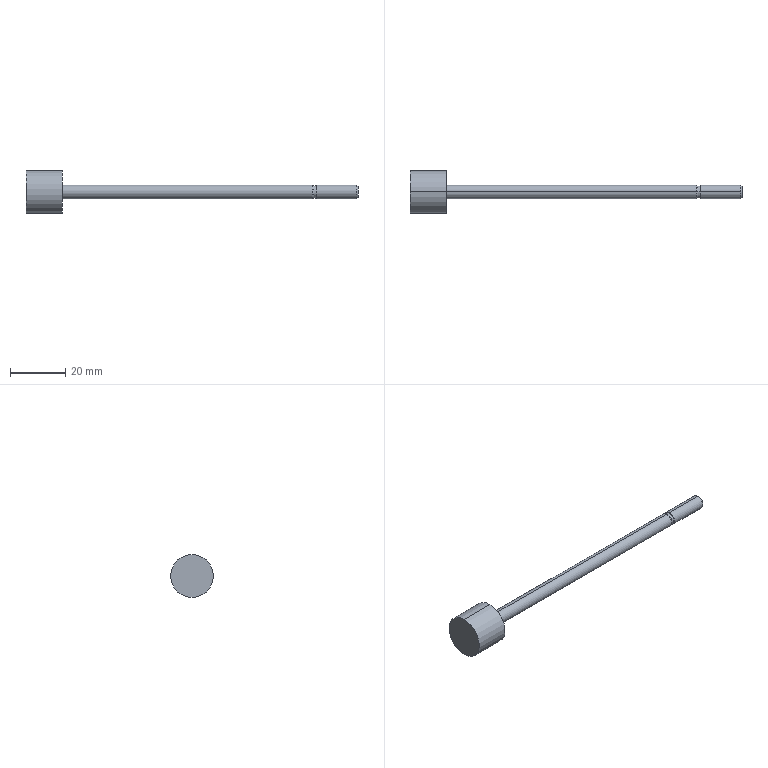Component | SolidWorks | 17268PB16x60SU(58)+(CS1-M-2)-1_1726816PB60URod-1 | 1 solid | 16 faces | box 120.36 x 15.5 x 15.5 mm | volume 4587 mm3 | cylinder 8 | cone 4 | plane 4 | commonest cylinder face diameters 5 x4 15.5 x2 4.38 x2
build123d program:
from build123d import *


with BuildPart() as part:
    # Sketch1 → Revolve1 (revolve)
    with BuildSketch(Plane.XY, mode=Mode.PRIVATE) as revolve1_sk:
        Polygon((0, 0), (0, 2.01), (0.4905, 2.5), (15, 2.5), (15, 2.19), (16, 2.19), (16.5, 2.5), (107.16, 2.5), (107.16, 7.75), (120.36, 7.75), (120.36, 0), align=None)
    revolve(revolve1_sk.sketch.rotate(Axis((120.36, 0, 0), (-1, 0, 0)), 270), axis=Axis((120.36, 0, 0), (-1, 0, 0)))


solid = part.part

# Placed as in the assembly
solid = solid.moved(Location((7, -27.579, 21.5), (-180, 0, 180)))
STEP:
#1=CARTESIAN_POINT('',(-4.463,-1.086,0.5413));
#2=VERTEX_POINT('',#1);
#3=CARTESIAN_POINT('',(-4.463,-1.086,1.152));
#4=VERTEX_POINT('',#3);
#5=CARTESIAN_POINT('',(-4.463,-1.086,0.8465));
#6=DIRECTION('',(1.,-0.,-0.));
#7=DIRECTION('',(0.,0.,-1.));
#8=AXIS2_PLACEMENT_3D('',#5,#6,#7);
#9=CIRCLE('',#8,0.3051);
#10=EDGE_CURVE('',#2,#4,#9,.T.);
#11=ORIENTED_EDGE('',*,*,#10,.T.);
#12=CARTESIAN_POINT('',(-3.943,-1.086,1.152));
#13=VERTEX_POINT('',#12);
#14=CARTESIAN_POINT('',(-4.463,-1.086,1.152));
#15=DIRECTION('',(1.,-0.,-0.));
#16=VECTOR('',#15,39.37);
#17=LINE('',#14,#16);
#18=EDGE_CURVE('',#4,#13,#17,.T.);
#19=ORIENTED_EDGE('',*,*,#18,.T.);
#20=CARTESIAN_POINT('',(-3.943,-1.086,0.5413));
#21=VERTEX_POINT('',#20);
#22=CARTESIAN_POINT('',(-3.943,-1.086,0.8465));
#23=DIRECTION('',(1.,-0.,-0.));
#24=DIRECTION('',(0.,0.,-1.));
#25=AXIS2_PLACEMENT_3D('',#22,#23,#24);
#26=CIRCLE('',#25,0.3051);
#27=EDGE_CURVE('',#21,#13,#26,.T.);
#28=ORIENTED_EDGE('',*,*,#27,.F.);
#29=CARTESIAN_POINT('',(-4.463,-1.086,0.5413));
#30=DIRECTION('',(1.,-0.,-0.));
#31=VECTOR('',#30,39.37);
#32=LINE('',#29,#31);
#33=EDGE_CURVE('',#2,#21,#32,.T.);
#34=ORIENTED_EDGE('',*,*,#33,.F.);
#35=EDGE_LOOP('',(#11,#19,#28,#34));
#36=FACE_OUTER_BOUND('',#35,.T.);
#37=CARTESIAN_POINT('',(-4.463,-1.086,0.8465));
#38=DIRECTION('',(1.,-0.,-0.));
#39=DIRECTION('',(0.,0.,-1.));
#40=AXIS2_PLACEMENT_3D('',#37,#38,#39);
#41=CYLINDRICAL_SURFACE('',#40,0.3051);
#42=ADVANCED_FACE('',(#36),#41,.T.);
#43=CARTESIAN_POINT('',(-3.943,-1.086,0.748));
#44=VERTEX_POINT('',#43);
#45=CARTESIAN_POINT('',(-3.943,-1.086,0.9449));
#46=VERTEX_POINT('',#45);
#47=CARTESIAN_POINT('',(-3.943,-1.086,0.8465));
#48=DIRECTION('',(1.,-0.,-0.));
#49=DIRECTION('',(0.,0.,-1.));
#50=AXIS2_PLACEMENT_3D('',#47,#48,#49);
#51=CIRCLE('',#50,0.09843);
#52=EDGE_CURVE('',#44,#46,#51,.T.);
#53=ORIENTED_EDGE('',*,*,#52,.T.);
#54=CARTESIAN_POINT('',(-0.374,-1.086,0.9449));
#55=VERTEX_POINT('',#54);
#56=CARTESIAN_POINT('',(-4.463,-1.086,0.9449));
#57=DIRECTION('',(1.,-0.,-0.));
#58=VECTOR('',#57,39.37);
#59=LINE('',#56,#58);
#60=EDGE_CURVE('',#46,#55,#59,.T.);
#61=ORIENTED_EDGE('',*,*,#60,.T.);
#62=CARTESIAN_POINT('',(-0.374,-1.086,0.748));
#63=VERTEX_POINT('',#62);
#64=CARTESIAN_POINT('',(-0.374,-1.086,0.8465));
#65=DIRECTION('',(1.,-0.,-0.));
#66=DIRECTION('',(0.,0.,-1.));
#67=AXIS2_PLACEMENT_3D('',#64,#65,#66);
#68=CIRCLE('',#67,0.09843);
#69=EDGE_CURVE('',#63,#55,#68,.T.);
#70=ORIENTED_EDGE('',*,*,#69,.F.);
#71=CARTESIAN_POINT('',(-4.463,-1.086,0.748));
#72=DIRECTION('',(1.,-0.,-0.));
#73=VECTOR('',#72,39.37);
#74=LINE('',#71,#73);
#75=EDGE_CURVE('',#44,#63,#74,.T.);
#76=ORIENTED_EDGE('',*,*,#75,.F.);
#77=EDGE_LOOP('',(#53,#61,#70,#76));
#78=FACE_OUTER_BOUND('',#77,.T.);
#79=CARTESIAN_POINT('',(-4.463,-1.086,0.8465));
#80=DIRECTION('',(1.,-0.,-0.));
#81=DIRECTION('',(0.,0.,-1.));
#82=AXIS2_PLACEMENT_3D('',#79,#80,#81);
#83=CYLINDRICAL_SURFACE('',#82,0.09843);
#84=ADVANCED_FACE('',(#78),#83,.T.);
#85=CARTESIAN_POINT('',(-0.3543,-1.086,0.7602));
#86=VERTEX_POINT('',#85);
#87=CARTESIAN_POINT('',(-0.3543,-1.086,0.9327));
#88=VERTEX_POINT('',#87);
#89=CARTESIAN_POINT('',(-0.3543,-1.086,0.8465));
#90=DIRECTION('',(1.,-0.,-0.));
#91=DIRECTION('',(0.,0.,-1.));
#92=AXIS2_PLACEMENT_3D('',#89,#90,#91);
#93=CIRCLE('',#92,0.08622);
#94=EDGE_CURVE('',#86,#88,#93,.T.);
#95=ORIENTED_EDGE('',*,*,#94,.F.);
#96=CARTESIAN_POINT('',(-0.374,-1.086,0.748));
#97=DIRECTION('',(-0.8499,0.,-0.5269));
#98=VECTOR('',#97,39.37);
#99=LINE('',#96,#98);
#100=EDGE_CURVE('',#86,#63,#99,.T.);
#101=ORIENTED_EDGE('',*,*,#100,.T.);
#102=ORIENTED_EDGE('',*,*,#69,.T.);
#103=CARTESIAN_POINT('',(-0.374,-1.086,0.9449));
#104=DIRECTION('',(-0.8499,0.,0.5269));
#105=VECTOR('',#104,39.37);
#106=LINE('',#103,#105);
#107=EDGE_CURVE('',#88,#55,#106,.T.);
#108=ORIENTED_EDGE('',*,*,#107,.F.);
#109=EDGE_LOOP('',(#95,#101,#102,#108));
#110=FACE_OUTER_BOUND('',#109,.T.);
#111=CARTESIAN_POINT('',(-0.374,-1.086,0.8465));
#112=DIRECTION('',(-1.,0.,0.));
#113=DIRECTION('',(0.,0.,1.));
#114=AXIS2_PLACEMENT_3D('',#111,#112,#113);
#115=CONICAL_SURFACE('',#114,0.09843,0.555);
#116=ADVANCED_FACE('',(#110),#115,.T.);
#117=ORIENTED_EDGE('',*,*,#94,.T.);
#118=CARTESIAN_POINT('',(-0.315,-1.086,0.9327));
#119=VERTEX_POINT('',#118);
#120=CARTESIAN_POINT('',(-4.463,-1.086,0.9327));
#121=DIRECTION('',(1.,-0.,-0.));
#122=VECTOR('',#121,39.37);
#123=LINE('',#120,#122);
#124=EDGE_CURVE('',#88,#119,#123,.T.);
#125=ORIENTED_EDGE('',*,*,#124,.T.);
#126=CARTESIAN_POINT('',(-0.315,-1.086,0.7602));
#127=VERTEX_POINT('',#126);
#128=CARTESIAN_POINT('',(-0.315,-1.086,0.8465));
#129=DIRECTION('',(1.,-0.,-0.));
#130=DIRECTION('',(0.,0.,-1.));
#131=AXIS2_PLACEMENT_3D('',#128,#129,#130);
#132=CIRCLE('',#131,0.08622);
#133=EDGE_CURVE('',#127,#119,#132,.T.);
#134=ORIENTED_EDGE('',*,*,#133,.F.);
#135=CARTESIAN_POINT('',(-4.463,-1.086,0.7602));
#136=DIRECTION('',(1.,-0.,-0.));
#137=VECTOR('',#136,39.37);
#138=LINE('',#135,#137);
#139=EDGE_CURVE('',#86,#127,#138,.T.);
#140=ORIENTED_EDGE('',*,*,#139,.F.);
#141=EDGE_LOOP('',(#117,#125,#134,#140));
#142=FACE_OUTER_BOUND('',#141,.T.);
#143=CARTESIAN_POINT('',(-4.463,-1.086,0.8465));
#144=DIRECTION('',(1.,-0.,-0.));
#145=DIRECTION('',(0.,0.,-1.));
#146=AXIS2_PLACEMENT_3D('',#143,#144,#145);
#147=CYLINDRICAL_SURFACE('',#146,0.08622);
#148=ADVANCED_FACE('',(#142),#147,.T.);
#149=CARTESIAN_POINT('',(-0.315,-1.086,0.748));
#150=VERTEX_POINT('',#149);
#151=CARTESIAN_POINT('',(-0.315,-1.086,0.9449));
#152=VERTEX_POINT('',#151);
#153=CARTESIAN_POINT('',(-0.315,-1.086,0.8465));
#154=DIRECTION('',(1.,-0.,-0.));
#155=DIRECTION('',(0.,0.,-1.));
#156=AXIS2_PLACEMENT_3D('',#153,#154,#155);
#157=CIRCLE('',#156,0.09843);
#158=EDGE_CURVE('',#150,#152,#157,.T.);
#159=ORIENTED_EDGE('',*,*,#158,.T.);
#160=CARTESIAN_POINT('',(0.2563,-1.086,0.9449));
#161=VERTEX_POINT('',#160);
#162=CARTESIAN_POINT('',(-4.463,-1.086,0.9449));
#163=DIRECTION('',(1.,-0.,-0.));
#164=VECTOR('',#163,39.37);
#165=LINE('',#162,#164);
#166=EDGE_CURVE('',#152,#161,#165,.T.);
#167=ORIENTED_EDGE('',*,*,#166,.T.);
#168=CARTESIAN_POINT('',(0.2563,-1.086,0.748));
#169=VERTEX_POINT('',#168);
#170=CARTESIAN_POINT('',(0.2563,-1.086,0.8465));
#171=DIRECTION('',(1.,-0.,-0.));
#172=DIRECTION('',(0.,0.,-1.));
#173=AXIS2_PLACEMENT_3D('',#170,#171,#172);
#174=CIRCLE('',#173,0.09843);
#175=EDGE_CURVE('',#169,#161,#174,.T.);
#176=ORIENTED_EDGE('',*,*,#175,.F.);
#177=CARTESIAN_POINT('',(-4.463,-1.086,0.748));
#178=DIRECTION('',(1.,-0.,-0.));
#179=VECTOR('',#178,39.37);
#180=LINE('',#177,#179);
#181=EDGE_CURVE('',#150,#169,#180,.T.);
#182=ORIENTED_EDGE('',*,*,#181,.F.);
#183=EDGE_LOOP('',(#159,#167,#176,#182));
#184=FACE_OUTER_BOUND('',#183,.T.);
#185=CARTESIAN_POINT('',(-4.463,-1.086,0.8465));
#186=DIRECTION('',(1.,-0.,-0.));
#187=DIRECTION('',(0.,0.,-1.));
#188=AXIS2_PLACEMENT_3D('',#185,#186,#187);
#189=CYLINDRICAL_SURFACE('',#188,0.09843);
#190=ADVANCED_FACE('',(#184),#189,.T.);
#191=CARTESIAN_POINT('',(0.2756,-1.086,0.7673));
#192=VERTEX_POINT('',#191);
#193=CARTESIAN_POINT('',(0.2756,-1.086,0.9256));
#194=VERTEX_POINT('',#193);
#195=CARTESIAN_POINT('',(0.2756,-1.086,0.8465));
#196=DIRECTION('',(1.,-0.,-0.));
#197=DIRECTION('',(0.,0.,-1.));
#198=AXIS2_PLACEMENT_3D('',#195,#196,#197);
#199=CIRCLE('',#198,0.07911);
#200=EDGE_CURVE('',#192,#194,#199,.T.);
#201=ORIENTED_EDGE('',*,*,#200,.F.);
#202=CARTESIAN_POINT('',(0.2563,-1.086,0.748));
#203=DIRECTION('',(-0.7071,0.,-0.7071));
#204=VECTOR('',#203,39.37);
#205=LINE('',#202,#204);
#206=EDGE_CURVE('',#192,#169,#205,.T.);
#207=ORIENTED_EDGE('',*,*,#206,.T.);
#208=ORIENTED_EDGE('',*,*,#175,.T.);
#209=CARTESIAN_POINT('',(0.2563,-1.086,0.9449));
#210=DIRECTION('',(-0.7071,0.,0.7071));
#211=VECTOR('',#210,39.37);
#212=LINE('',#209,#211);
#213=EDGE_CURVE('',#194,#161,#212,.T.);
#214=ORIENTED_EDGE('',*,*,#213,.F.);
#215=EDGE_LOOP('',(#201,#207,#208,#214));
#216=FACE_OUTER_BOUND('',#215,.T.);
#217=CARTESIAN_POINT('',(0.2563,-1.086,0.8465));
#218=DIRECTION('',(-1.,0.,0.));
#219=DIRECTION('',(0.,0.,1.));
#220=AXIS2_PLACEMENT_3D('',#217,#218,#219);
#221=CONICAL_SURFACE('',#220,0.09843,0.7854);
#222=ADVANCED_FACE('',(#216),#221,.T.);
#223=CARTESIAN_POINT('',(0.2756,-1.086,0.8465));
#224=DIRECTION('',(1.,-0.,-0.));
#225=DIRECTION('',(0.,0.,-1.));
#226=AXIS2_PLACEMENT_3D('',#223,#224,#225);
#227=CIRCLE('',#226,0.07911);
#228=EDGE_CURVE('',#194,#192,#227,.T.);
#229=ORIENTED_EDGE('',*,*,#228,.T.);
#230=ORIENTED_EDGE('',*,*,#200,.T.);
#231=EDGE_LOOP('',(#229,#230));
#232=FACE_OUTER_BOUND('',#231,.T.);
#233=CARTESIAN_POINT('',(0.2756,-1.086,0.8465));
#234=DIRECTION('',(-1.,0.,0.));
#235=DIRECTION('',(0.,0.,1.));
#236=AXIS2_PLACEMENT_3D('',#233,#234,#235);
#237=PLANE('',#236);
#238=ADVANCED_FACE('',(#232),#237,.F.);
#239=ORIENTED_EDGE('',*,*,#206,.F.);
#240=ORIENTED_EDGE('',*,*,#228,.F.);
#241=ORIENTED_EDGE('',*,*,#213,.T.);
#242=CARTESIAN_POINT('',(0.2563,-1.086,0.8465));
#243=DIRECTION('',(1.,-0.,-0.));
#244=DIRECTION('',(0.,0.,-1.));
#245=AXIS2_PLACEMENT_3D('',#242,#243,#244);
#246=CIRCLE('',#245,0.09843);
#247=EDGE_CURVE('',#161,#169,#246,.T.);
#248=ORIENTED_EDGE('',*,*,#247,.T.);
#249=EDGE_LOOP('',(#239,#240,#241,#248));
#250=FACE_OUTER_BOUND('',#249,.T.);
#251=CARTESIAN_POINT('',(0.2563,-1.086,0.8465));
#252=DIRECTION('',(-1.,0.,0.));
#253=DIRECTION('',(0.,0.,1.));
#254=AXIS2_PLACEMENT_3D('',#251,#252,#253);
#255=CONICAL_SURFACE('',#254,0.09843,0.7854);
#256=ADVANCED_FACE('',(#250),#255,.T.);
#257=ORIENTED_EDGE('',*,*,#166,.F.);
#258=CARTESIAN_POINT('',(-0.315,-1.086,0.8465));
#259=DIRECTION('',(1.,-0.,-0.));
#260=DIRECTION('',(0.,0.,-1.));
#261=AXIS2_PLACEMENT_3D('',#258,#259,#260);
#262=CIRCLE('',#261,0.09843);
#263=EDGE_CURVE('',#152,#150,#262,.T.);
#264=ORIENTED_EDGE('',*,*,#263,.T.);
#265=ORIENTED_EDGE('',*,*,#181,.T.);
#266=ORIENTED_EDGE('',*,*,#247,.F.);
#267=EDGE_LOOP('',(#257,#264,#265,#266));
#268=FACE_OUTER_BOUND('',#267,.T.);
#269=CARTESIAN_POINT('',(-4.463,-1.086,0.8465));
#270=DIRECTION('',(1.,-0.,-0.));
#271=DIRECTION('',(0.,0.,-1.));
#272=AXIS2_PLACEMENT_3D('',#269,#270,#271);
#273=CYLINDRICAL_SURFACE('',#272,0.09843);
#274=ADVANCED_FACE('',(#268),#273,.T.);
#275=ORIENTED_EDGE('',*,*,#158,.F.);
#276=ORIENTED_EDGE('',*,*,#263,.F.);
#277=EDGE_LOOP('',(#275,#276));
#278=FACE_OUTER_BOUND('',#277,.T.);
#279=ORIENTED_EDGE('',*,*,#133,.T.);
#280=CARTESIAN_POINT('',(-0.315,-1.086,0.8465));
#281=DIRECTION('',(1.,-0.,-0.));
#282=DIRECTION('',(0.,0.,-1.));
#283=AXIS2_PLACEMENT_3D('',#280,#281,#282);
#284=CIRCLE('',#283,0.08622);
#285=EDGE_CURVE('',#119,#127,#284,.T.);
#286=ORIENTED_EDGE('',*,*,#285,.T.);
#287=EDGE_LOOP('',(#279,#286));
#288=FACE_BOUND('',#287,.T.);
#289=CARTESIAN_POINT('',(-0.315,-0.9874,0.8465));
#290=DIRECTION('',(1.,-0.,-0.));
#291=DIRECTION('',(-0.,0.,-1.));
#292=AXIS2_PLACEMENT_3D('',#289,#290,#291);
#293=PLANE('',#292);
#294=ADVANCED_FACE('',(#278,#288),#293,.F.);
#295=ORIENTED_EDGE('',*,*,#124,.F.);
#296=CARTESIAN_POINT('',(-0.3543,-1.086,0.8465));
#297=DIRECTION('',(1.,-0.,-0.));
#298=DIRECTION('',(0.,0.,-1.));
#299=AXIS2_PLACEMENT_3D('',#296,#297,#298);
#300=CIRCLE('',#299,0.08622);
#301=EDGE_CURVE('',#88,#86,#300,.T.);
#302=ORIENTED_EDGE('',*,*,#301,.T.);
#303=ORIENTED_EDGE('',*,*,#139,.T.);
#304=ORIENTED_EDGE('',*,*,#285,.F.);
#305=EDGE_LOOP('',(#295,#302,#303,#304));
#306=FACE_OUTER_BOUND('',#305,.T.);
#307=CARTESIAN_POINT('',(-4.463,-1.086,0.8465));
#308=DIRECTION('',(1.,-0.,-0.));
#309=DIRECTION('',(0.,0.,-1.));
#310=AXIS2_PLACEMENT_3D('',#307,#308,#309);
#311=CYLINDRICAL_SURFACE('',#310,0.08622);
#312=ADVANCED_FACE('',(#306),#311,.T.);
#313=ORIENTED_EDGE('',*,*,#100,.F.);
#314=ORIENTED_EDGE('',*,*,#301,.F.);
#315=ORIENTED_EDGE('',*,*,#107,.T.);
#316=CARTESIAN_POINT('',(-0.374,-1.086,0.8465));
#317=DIRECTION('',(1.,-0.,-0.));
#318=DIRECTION('',(0.,0.,-1.));
#319=AXIS2_PLACEMENT_3D('',#316,#317,#318);
#320=CIRCLE('',#319,0.09843);
#321=EDGE_CURVE('',#55,#63,#320,.T.);
#322=ORIENTED_EDGE('',*,*,#321,.T.);
#323=EDGE_LOOP('',(#313,#314,#315,#322));
#324=FACE_OUTER_BOUND('',#323,.T.);
#325=CARTESIAN_POINT('',(-0.374,-1.086,0.8465));
#326=DIRECTION('',(-1.,0.,0.));
#327=DIRECTION('',(0.,0.,1.));
#328=AXIS2_PLACEMENT_3D('',#325,#326,#327);
#329=CONICAL_SURFACE('',#328,0.09843,0.555);
#330=ADVANCED_FACE('',(#324),#329,.T.);
#331=ORIENTED_EDGE('',*,*,#60,.F.);
#332=CARTESIAN_POINT('',(-3.943,-1.086,0.8465));
#333=DIRECTION('',(1.,-0.,-0.));
#334=DIRECTION('',(0.,0.,-1.));
#335=AXIS2_PLACEMENT_3D('',#332,#333,#334);
#336=CIRCLE('',#335,0.09843);
#337=EDGE_CURVE('',#46,#44,#336,.T.);
#338=ORIENTED_EDGE('',*,*,#337,.T.);
#339=ORIENTED_EDGE('',*,*,#75,.T.);
#340=ORIENTED_EDGE('',*,*,#321,.F.);
#341=EDGE_LOOP('',(#331,#338,#339,#340));
#342=FACE_OUTER_BOUND('',#341,.T.);
#343=CARTESIAN_POINT('',(-4.463,-1.086,0.8465));
#344=DIRECTION('',(1.,-0.,-0.));
#345=DIRECTION('',(0.,0.,-1.));
#346=AXIS2_PLACEMENT_3D('',#343,#344,#345);
#347=CYLINDRICAL_SURFACE('',#346,0.09843);
#348=ADVANCED_FACE('',(#342),#347,.T.);
#349=ORIENTED_EDGE('',*,*,#52,.F.);
#350=ORIENTED_EDGE('',*,*,#337,.F.);
#351=EDGE_LOOP('',(#349,#350));
#352=FACE_BOUND('',#351,.T.);
#353=ORIENTED_EDGE('',*,*,#27,.T.);
#354=CARTESIAN_POINT('',(-3.943,-1.086,0.8465));
#355=DIRECTION('',(1.,-0.,-0.));
#356=DIRECTION('',(0.,0.,-1.));
#357=AXIS2_PLACEMENT_3D('',#354,#355,#356);
#358=CIRCLE('',#357,0.3051);
#359=EDGE_CURVE('',#13,#21,#358,.T.);
#360=ORIENTED_EDGE('',*,*,#359,.T.);
#361=EDGE_LOOP('',(#353,#360));
#362=FACE_OUTER_BOUND('',#361,.T.);
#363=CARTESIAN_POINT('',(-3.943,-0.9874,0.8465));
#364=DIRECTION('',(-1.,0.,0.));
#365=DIRECTION('',(0.,0.,1.));
#366=AXIS2_PLACEMENT_3D('',#363,#364,#365);
#367=PLANE('',#366);
#368=ADVANCED_FACE('',(#352,#362),#367,.F.);
#369=ORIENTED_EDGE('',*,*,#18,.F.);
#370=CARTESIAN_POINT('',(-4.463,-1.086,0.8465));
#371=DIRECTION('',(1.,-0.,-0.));
#372=DIRECTION('',(0.,0.,-1.));
#373=AXIS2_PLACEMENT_3D('',#370,#371,#372);
#374=CIRCLE('',#373,0.3051);
#375=EDGE_CURVE('',#4,#2,#374,.T.);
#376=ORIENTED_EDGE('',*,*,#375,.T.);
#377=ORIENTED_EDGE('',*,*,#33,.T.);
#378=ORIENTED_EDGE('',*,*,#359,.F.);
#379=EDGE_LOOP('',(#369,#376,#377,#378));
#380=FACE_OUTER_BOUND('',#379,.T.);
#381=CARTESIAN_POINT('',(-4.463,-1.086,0.8465));
#382=DIRECTION('',(1.,-0.,-0.));
#383=DIRECTION('',(0.,0.,-1.));
#384=AXIS2_PLACEMENT_3D('',#381,#382,#383);
#385=CYLINDRICAL_SURFACE('',#384,0.3051);
#386=ADVANCED_FACE('',(#380),#385,.T.);
#387=ORIENTED_EDGE('',*,*,#10,.F.);
#388=ORIENTED_EDGE('',*,*,#375,.F.);
#389=EDGE_LOOP('',(#387,#388));
#390=FACE_OUTER_BOUND('',#389,.T.);
#391=CARTESIAN_POINT('',(-4.463,-0.7807,0.8465));
#392=DIRECTION('',(1.,-0.,-0.));
#393=DIRECTION('',(-0.,0.,-1.));
#394=AXIS2_PLACEMENT_3D('',#391,#392,#393);
#395=PLANE('',#394);
#396=ADVANCED_FACE('',(#390),#395,.F.);
#397=CLOSED_SHELL('',(#42,#84,#116,#148,#190,#222,#238,#256,#274,#294,#312,#330,#348,#368,#386,#396));
#398=MANIFOLD_SOLID_BREP('',#397);
#399=CARTESIAN_POINT('',(0.,0.,0.));
#400=DIRECTION('',(0.,0.,1.));
#401=DIRECTION('',(1.,0.,0.));
#402=AXIS2_PLACEMENT_3D('',#399,#400,#401);
#403=(LENGTH_UNIT()NAMED_UNIT(*)SI_UNIT($,.METRE.));
#404=LENGTH_MEASURE_WITH_UNIT(LENGTH_MEASURE(0.0254),#403);
#405=DIMENSIONAL_EXPONENTS(1.,0.,0.,0.,0.,0.,0.);
#406=(CONVERSION_BASED_UNIT('',#404)LENGTH_UNIT()NAMED_UNIT(#405));
#407=UNCERTAINTY_MEASURE_WITH_UNIT(LENGTH_MEASURE(0.00001),#406,'','');
#408=(NAMED_UNIT(*)PLANE_ANGLE_UNIT()SI_UNIT($,.RADIAN.));
#409=(NAMED_UNIT(*)SI_UNIT($,.STERADIAN.)SOLID_ANGLE_UNIT());
#410=(GEOMETRIC_REPRESENTATION_CONTEXT(3)GLOBAL_UNCERTAINTY_ASSIGNED_CONTEXT((#407))GLOBAL_UNIT_ASSIGNED_CONTEXT((#406,#408,#409))REPRESENTATION_CONTEXT('',''));
#411=ADVANCED_BREP_SHAPE_REPRESENTATION('',(#398,#402),#410);
#412=COLOUR_RGB('',0.7922,0.8196,0.9333);
#413=FILL_AREA_STYLE_COLOUR('',#412);
#414=FILL_AREA_STYLE('',(#413));
#415=SURFACE_STYLE_FILL_AREA(#414);
#416=SURFACE_SIDE_STYLE('',(#415));
#417=SURFACE_STYLE_USAGE(.BOTH.,#416);
#418=PRESENTATION_STYLE_ASSIGNMENT((#417));
#419=STYLED_ITEM('',(#418),#398);
#420=PRESENTATION_LAYER_ASSIGNMENT('','',(#419));
#421=(LENGTH_UNIT()NAMED_UNIT(*)SI_UNIT($,.METRE.));
#422=LENGTH_MEASURE_WITH_UNIT(LENGTH_MEASURE(0.0254),#421);
#423=DIMENSIONAL_EXPONENTS(1.,0.,0.,0.,0.,0.,0.);
#424=(CONVERSION_BASED_UNIT('',#422)LENGTH_UNIT()NAMED_UNIT(#423));
#425=UNCERTAINTY_MEASURE_WITH_UNIT(LENGTH_MEASURE(0.00001),#424,'','');
#426=(NAMED_UNIT(*)PLANE_ANGLE_UNIT()SI_UNIT($,.RADIAN.));
#427=(NAMED_UNIT(*)SI_UNIT($,.STERADIAN.)SOLID_ANGLE_UNIT());
#428=(GEOMETRIC_REPRESENTATION_CONTEXT(3)GLOBAL_UNCERTAINTY_ASSIGNED_CONTEXT((#425))GLOBAL_UNIT_ASSIGNED_CONTEXT((#424,#426,#427))REPRESENTATION_CONTEXT('',''));
#429=MECHANICAL_DESIGN_GEOMETRIC_PRESENTATION_REPRESENTATION('',(#419),#428);